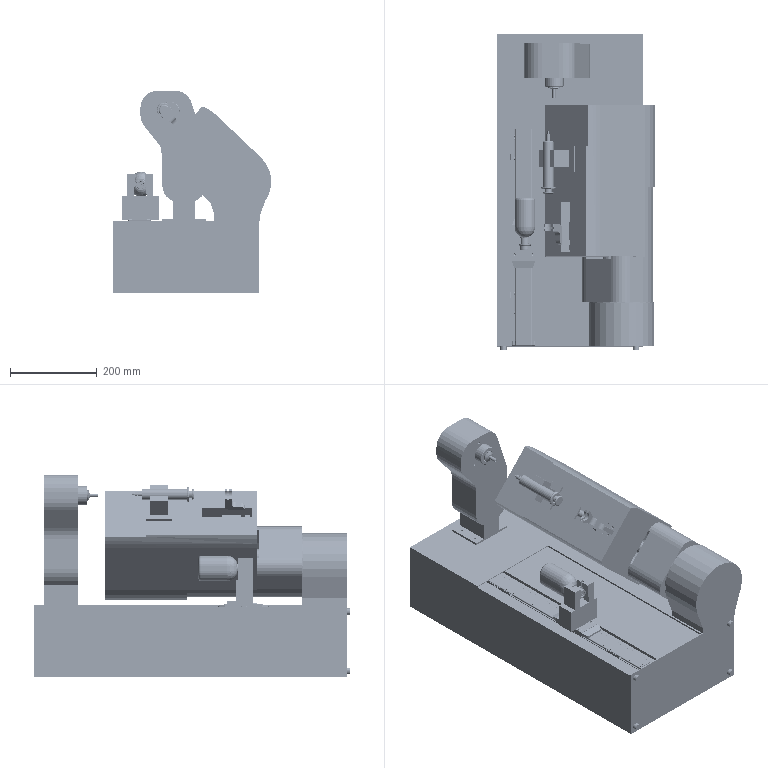Assembly | SolidWorks | mm | 70 component files | 94 solids | 5517 faces | box 364.9 x 728 x 466.99 mm | volume 10664747 mm3 | plane 2518 | cylinder 1839 | cone 608 | torus 290 | spline 142 | sphere 120 | commonest cylinder face diameters 4 x124 3.3 x122 8 x92 2 x85 4.5 x66 3 x64 5.5 x62 6 x61
Bill of materials:
1 | 1 |  | Long straight prismatic extrusion with a rectangular, double-cell slotted cross-section; looks like a T-slot framing profile.
circlips for shaft--type a small gb_GB_CONNECTING_PIECE_RING_RRA 8 | 1 |  | Thin flat open ring with a lobe on one side. A radial split passes through the lobe and has a small circular cutout across it.
Copy(10) | 1 |  | Cylindrical part made of two end hubs and a middle section with interlocking jaw or tooth blocks. It has an axial bore, and one end has a radial clamp slit. Resembles a jaw-type shaft coupling.
Copy(11) | 1 |  | Housing with a square body and a square front flange, a circular pilot boss, and a protruding cylindrical shaft with a keyway or flat. Resembles a rotary motor envelope.
Copy(2) | 1 |  | Flanged cylindrical sleeve with a through bore. The circular flange has two straight flats and six bolt holes. Resembles a flanged nut or bushing.
Copy(3) | 1 |  | Stepped cylindrical shaft: a long main diameter with reduced-diameter journals at both ends. One end has a longer journal; the other has a short double step.
Copy(4) | 1 |  | Long straight rail with a profiled cross-section, side grooves and a row of evenly spaced vertical counterbored holes along its length. Resembles a linear guide rail.
Copy(5) | 1 |  | Rectangular block with an inverted-channel underside shaped to straddle a rail, four mounting holes on top, and end caps or plates. Resembles a linear guide carriage.
Copy(6) | 1 |  | Rectangular block with a large through bore, several groups of small holes on different faces, and a shallow step or rebate along one lower edge.
Copy(7) | 1 |  | L-shaped bracket. The upright plate carries a large through hole; the base leg has two counterbored mounting holes. Resembles a shaft or bearing support bracket.
Copy(8) | 1 |  | Flat rectangular plate with one rounded corner, one large through hole near one end and two small through holes near the opposite end.
Copy(9) | 1 |  | Flat rectangular plate with one rounded corner, a large central through hole and six smaller holes of two sizes. Possibly a mounting or adapter plate.
deep groove ball bearings gb_Rolling bearings 608 GB 276-94 | 2 |  | Ring-shaped assembly that looks like a radial ball bearing: a concentric outer ring and inner ring with a row of spherical balls between them.
hex nuts, style 1-grades ab gb_GB_FASTENER_NUT_SNAB1 M4-N | 2 |  | Hexagonal nut-like prism with a central cylindrical through-bore and chamfered corners on both faces.
hexagon socket head cap screws gb_GB_FASTENER_SCREWS_HSHCS M3X8-N | 7 |  | Cap-screw-like fastener: a cylindrical head with a hexagonal socket recess and a plain cylindrical shank with a chamfered tip.
hexagon socket head cap screws gb_GB_FASTENER_SCREWS_HSHCS M4X16-N | 4 |  | Headed pin or screw-like part: a cylindrical head with a rounded top edge and a long, slender plain cylindrical shank with a chamfered end.
hexagon socket head cap screws gb_GB_FASTENER_SCREWS_HSHCS M4X8-N | 2 |  | Short cap-screw-like fastener: a cylindrical head with a hexagonal socket and a short plain cylindrical shank.
20mL - Glass Barrel | 1 | Glass | Long hollow cylindrical barrel. One end has a flange with flats; the other end has a stepped, narrow nozzle-like tip with a small axial hole. The shape resembles a syringe or cartridge barrel.
20mL - Glass Syringe Plunger | 1 | Glass | Solid stepped cylindrical rod: a thin disc-shaped end flange, a short reduced-diameter neck, and a long main cylinder with a chamfered far end. The shape resembles a plunger.
InjectionFixture | 1 |  | Prismatic block with a stepped outline, a semicircular cutout on one side and a thin plate-like flange along one edge.
_GTH5.-BC_body6^3359524133GTH5-400-BC(2) | 1 |  | Block-shaped bracket or housing: a rectangular body with a curved saddle-like channel across its top, and a thin back plate with two small holes and a larger circular opening.
GTH4-sensor_plant | 3 |  | L-shaped bent sheet-metal-style bracket. The horizontal flange has two open slots and four round holes; the vertical flange carries two stepped cylindrical pins.
GTH4-sensor | 3 |  | Rectangular body with two upright prongs that form an open U-shaped slot, an elongated base, a cylindrical rod or cable stub out one end, and a mounting tab with a small cylindrical boss. The shape resembles a slot-type sensor package.
GTH5_body3 | 1 |  | Flat plate with a T-shaped outline and rounded edges. It has a wider lower section with four counterbored holes and a narrower upper section with a step or groove near its top edge.
GTH5_body4 | 1 |  | Thick, nearly square plate with one large central circular through-hole that has a stepped/counterbored edge, and four small through-holes in two pairs near the lower corners.
GTH5-400-BC_body | 1 |  | Long straight extruded-profile body with a stepped cross-section: a wide lower base and a narrower upper section with slots along both sides near the top, end plates/caps with small fasteners, and a row of evenly spaced small holes along the length.
GTH5-400-BC_body2 | 1 |  | Very thin, long, narrow flat strip with two small holes at each end.
GTH5-400-BC_slider | 1 |  | Flat, rectangular carriage-like plate with tapered (chamfered-outline) end sections, a pattern of counterbored holes and socket-head-like fastener features on top, raised pads, and a small cylindrical stub sticking out of one side.
GTH5-50-BC_slider2 | 1 |  | Bent flat-bar bracket with a Z or joggled profile: two parallel offset legs joined by a short perpendicular web. One leg has two round through-holes.
GTH5-BC_body5 | 1 |  | U-shaped (inverted channel) cover made from a thin wall, with raised embossed lettering on the top face and a small circular boss or hole on one side wall.
M10-p1 | 1 |  | Compact rectangular block body made of several stacked segments, including one tapered section. A stepped cylindrical shaft sticks out of one face from a rectangular boss, there is a second short cylindrical stub, and a rounded rib runs along one edge.
ArmHousing | 1 |  | Solid prismatic extrusion with a keyhole/bulb-shaped profile: a circular arc top that narrows into tapered flanks and ends in a short rectangular base.
ArmHousing2 | 1 |  | Very thin flat plate with the same bulb/keyhole outline as a rounded tab: a circular top with a large concentric round hole, tapered sides, and a straight rectangular foot.
ArmHousing3 | 1 |  | Long solid prism with a rounded, teardrop/rounded-triangular cross-section. One end face has a central round hole surrounded by a ring of small holes.
DAS-15SS^ClampBlock | 1 |  | Stepped cylindrical body: a larger-diameter flange section with three axial through-holes and a smaller-diameter tubular spigot with a central bore. Two hex-bodied fittings stick out radially from the flange periphery, and there are small radial holes in the spigot.
YB-15^ClampBlock | 1 |  | Collet-like cylindrical part: a tapered head with an outward cone, three longitudinal slots splitting the head end, a central bore, plain cylindrical bands, and an externally threaded end.
FlatJawHousing | 1 |  | Thin flat plate with a bent, elongated outline: a wide rounded upper lobe angled to one side, a straighter lower section, and a narrow neck that ends in a thin T-shaped foot strip.
Housing | 1 |  | Rectangular box-shaped solid. The top face has a long recessed channel along one edge, a stepped panel line, small holes, and a stepped notch cutout at one corner. Short cylindrical studs stick out from one end face.
InjectionRodClamp | 1 |  | Bent bracket arm with an S-shaped joggle. One end is a forked or slotted tip with a semicircular notch. The other end is a rectangular mounting block with four through holes.
LiquidReagentBottle | 1 |  | Bottle-like solid of revolution: a cylindrical body with a rounded closed end, a curved shoulder, and a stepped neck with a raised collar. The end face carries concentric rings and two small circular features.
MotorHousing | 1 |  | Thin-walled shell with a D-shaped or U-shaped cross section: flat sides joined by a semicircular end. It has an offset stepped section and a rectangular window or slot in one side wall.
NeedleClampBlock | 1 |  | Thick block with the same bent, elongated outline as a lobed plate. The upper lobe has a large circular through bore with three small holes around it. A narrower neck stands on a thin base plate that has small holes.
NeedleSleeve | 1 |  | Stepped cylindrical tube: a longer section with a larger outside diameter and a shorter section with a smaller one. One end is open with a visible bore.
100Travel3872-3DDrawing | 1 |  | Housing with two parallel cylinders: a shorter cylinder and a longer main tube, joined at one end by a rounded housing block. A short tab with a cross hole sticks out from that end.
Axis | 1 |  | Slender, straight solid cylindrical rod, rendered dark. There may be small cross holes near the ends.
PushRodMotorPlatform | 1 |  | Flat circular disc with a smaller raised concentric step on one face, a central through hole, and a ring of twelve small holes around the centre. Two of the ring holes look slightly larger.
ReagentBottleClampBlock | 1 |  | Rectangular base block with two upright posts separated by a gap with curved, tapering walls. The post tops have notches. One face has two round holes, and there is a small stepped ledge at one side.
Base | 1 | 45 | Square block with chamfered corners, a central through bore, and four corner holes on the main face. A circular boss or pilot sticks out from the back. The stepped side faces carry several holes, some of which appear countersunk.
EE_SX672 | 1 |  | Rectangular block housing with an open U-shaped slot that splits it into two parallel arms. It has a pair of side mounting flanges with obround holes and four flat tab terminals, each with a round hole, along one end.
hexagon socket button head screws gb | 2 |  | Solid round shank with a dome-shaped (round) head at one end and a flat, plain end at the other.
InductionPlate | 1 | 45 | Bent flat strip shaped as a 90-degree L-bracket. It has a short top leg and a longer leg with rounded lower corners and two round through-holes.
PlanetaryReducer | 1 | 45 | Body with a square flange and a protruding cylindrical shaft. It has a square mounting flange with four corner holes, a round raised boss (pilot) around the shaft, a body with lengthwise recessed channels, and a wider square base with chamfered corners.
Turntable | 1 | 45 | Stepped cylindrical bushing with a central through-hole, a larger-diameter flange at one end, and a rectangular notch cut into the flange rim.
Mates:
1. coincident | 3359524133GTH5-400-BC(2)-1/GTH5-400-BC_slider-1 face at (334.847, 1139.269, -2179.834) dir (0, 0, 1) | ReagentBottleClampBlock-1 face at (362.347, 1094.769, -2179.834) dir (0, 0, -1)
2. distance | 3359524133GTH5-400-BC(2)-1/GTH5-400-BC_slider-1 face at (334.847, 1139.769, -2181.334) dir (0, 1, 0) | ReagentBottleClampBlock-1 face at (392.347, 1114.769, -2124.834) dir (0, 1, 0)
3. distance | ReagentBottleClampBlock-1 face at (319.847, 1074.769, -2179.834) dir (-1, 0, 0) | 3359524133GTH5-400-BC(2)-1/GTH5-400-BC_slider-1 face at (334.847, 1139.769, -2179.334) dir (-1, 0, 0)
4. lock | ReagentBottleClampBlock-1 reference at (0, 0, 0) dir (1, 0, 0) | LiquidReagentBottle-1 reference at (0, 0, 0) dir (1, 0, 0)
5. concentric | ArmHousing-1 face at (586.439, 647.868, -2092.934) dir (0, 1, 0) r 73 | RR40-1/Base-1 face at (586.439, 948, -2092.934) dir (0, -1, 0) r 47.5
6. distance | ArmHousing-1 face at (365.049, 960, -2167.934) dir (0, 1, 0) | RR40-1/InductionPlate-1 face at (594.447, 958, -2063.065) dir (0, 1, 0)
7. coincident | ArmHousing-1 edge at (586.439, 960, -2092.934) dir (0, 1, 0) r 75 | ArmHousing2-1 edge at (586.439, 960, -2092.934) dir (0, 1, 0) r 75
8. coincident | Housing-1 face at (129.525, 1580, -2182.934) dir (0, 0, 1) | ArmHousing-1 face at (365.049, 1412, -2182.934) dir (0, 0, -1)
9. coincident | Housing-1 face at (299.537, 860, -2241.334) dir (0, -1, 0) | ArmHousing-1 face at (365.049, 860, -2167.934) dir (0, -1, 0)
10. coincident | ArmHousing-1 edge at (533.489, 960, -2182.934) dir (1, 0, 0) | ArmHousing2-1 edge at (639.388, 960, -2182.934) dir (-1, 0, 0)
11. concentric | ArmHousing-1 face at (586.439, 647.868, -2092.934) dir (0, 1, 0) r 75 | ArmHousing3-1 face at (586.439, 1312, -2092.934) dir (0, -1, 0) r 73
12. parallel | Housing-1 face at (299.537, 860, -2241.334) dir (-1, 0, 0) | RR40-1/PlanetaryReducer-1 face at (564.439, 929.394, -2176.934) dir (-1, 0, 0)
13. coincident | ArmHousing2-1 face at (586.439, 962, -2092.934) dir (0, 1, 0) | ArmHousing3-1 face at (586.439, 962, -2092.934) dir (0, -1, 0)
14. parallel | ArmHousing2-1 face at (586.439, 962, -2092.934) dir (0, 1, 0) | MotorHousing-1 face at (584.807, 1067, -2032.144) dir (0, -1, 0)
15. parallel | ArmHousing3-1 face at (483.238, 1312, -2095.704) dir (-0.7258, 0, 0.6879) | 100-1/Copy(8)-1 face at (519.079, 1072, -2057.886) dir (0.7258, 0, -0.6879)
16. coincident | ArmHousing3-1 face at (483.238, 1312, -2095.704) dir (-0.7258, 0, 0.6879) | 100-1/Copy(8)-1 face at (519.079, 1072, -2057.886) dir (0.7258, 0, -0.6879)
17. concentric | ArmHousing3-1 face at (615.297, 964, -2105.562) dir (0, -1, 0) r 1.65 | PushRodMotorPlatform-1 face at (615.297, 976, -2105.562) dir (0, -1, 0) r 1.65
18. concentric | ArmHousing3-1 face at (557.104, 964, -2104.41) dir (0, -1, 0) r 1.65 | PushRodMotorPlatform-1 face at (557.104, 976, -2104.41) dir (0, -1, 0) r 1.65
19. concentric | ArmHousing3-1 face at (586.439, 1312, -2092.934) dir (0, -1, 0) r 73 | MotorHousing-1 face at (586.439, 1427, -2092.934) dir (0, -1, 0) r 78
20. coincident | PushRodMotorPlatform-1 face at (586.439, 976, -2092.934) dir (0, 1, 0) | PushRodMotor-1/100Travel3872-3DDrawing-1 face at (588.412, 976, -2097.251) dir (0, -1, 0)
21. lock | PushRodMotorPlatform-1 reference at (0, 0, 0) dir (1, 0, 0) | PushRodMotor-1/100Travel3872-3DDrawing-1 reference at (0, 0, 0) dir (1, 0, 0)
22. coincident | PushRodMotor-1/Axis-1 face at (588.412, 1411.001, -2097.251) dir (0, 1, 0) | MotorHousing-1 face at (482.645, 1411.001, -1994.567) dir (0, -1, 0)
23. coincident | MotorHousing-1 face at (512.224, 1072, -1963.357) dir (0, 1, 0) | 100-1/Copy(8)-1 face at (509.935, 1072, -2020.287) dir (0, -1, 0)
24. lock | MotorHousing-1 reference at (0, 0, 0) dir (1, 0, 0) | 100-1/Copy(8)-1 reference at (0, 0, 0) dir (1, 0, 0)
25. coincident | MotorHousing-1 face at (409.292, 860.697, -2021.086) dir (-0.7258, 0, 0.6879) | 20mL - Glass Syringe-1/InjectionFixture-1 face at (459.791, 1332, -1967.801) dir (0.7258, 0, -0.6879)
26. parallel | MotorHousing-1 face at (584.807, 1067, -2032.144) dir (0, -1, 0) | 20mL - Glass Syringe-1/InjectionFixture-1 face at (480.427, 1322, -1946.026) dir (0, 1, 0)
27. distance | 20mL - Glass Syringe-1/InjectionFixture-1 face at (480.427, 1262, -1946.026) dir (0.6879, 0, 0.7258) | MotorHousing-1 edge at (505.191, 1067, -1919.897) dir (0, 1, 0)
28. coincident | MotorHousing-1 face at (482.645, 1322, -1994.567) dir (0, 1, 0) | 20mL - Glass Syringe-1/InjectionFixture-1 face at (480.427, 1322, -1946.026) dir (0, 1, 0)
29. concentric | 100-1/Copy(6)-1 face at (489.45, 1091.461, -1987.096) dir (-0.7258, 0, 0.6879) r 3 | InjectionRodClamp-1 face at (485.821, 1091.461, -1983.657) dir (0.7258, 0, -0.6879) r 3
30. coincident | 100-1/Copy(6)-1 face at (499.081, 1146.461, -1976.934) dir (-0.7258, 0, 0.6879) | InjectionRodClamp-1 edge at (470.534, 1086.461, -2007.056) dir (0.6879, 0, 0.7258)
31. concentric | 100-1/Copy(6)-1 face at (475.693, 1106.461, -2001.613) dir (-0.7258, 0, 0.6879) r 3 | InjectionRodClamp-1 face at (472.064, 1106.461, -1998.173) dir (0.7258, 0, -0.6879) r 3
32. coincident | NeedleClampBlock-1 face at (431.234, 1505.5, -1930.507) dir (0, 1, 0) | ClampBlock-1/DAS-15SS^ClampBlock-1 face at (421.906, 1505.5, -1894.186) dir (0, -1, 0)
33. concentric | NeedleClampBlock-1 face at (431.234, 1577.5, -1930.507) dir (0, -1, 0) r 37.5 | ClampBlock-1/DAS-15SS^ClampBlock-1 face at (431.234, 1547.5, -1930.507) dir (0, 1, 0) r 37.5
34. concentric | ClampBlock-1/DAS-15SS^ClampBlock-1 face at (431.234, 1547.5, -1930.507) dir (0, 1, 0) r 22 | NeedleSleeve-1 face at (431.234, 1462, -1930.507) dir (0, -1, 0) r 4
35. distance | NeedleSleeve-1 face at (431.234, 1432, -1930.507) dir (0, -1, 0) | ClampBlock-1/YB-15^ClampBlock-1 face at (429.741, 1452, -1924.696) dir (0, -1, 0)
36. lock | Copy(2)-1 reference at (0, 0, 0) dir (1, 0, 0) | Copy(6)-1 reference at (0, 0, 0) dir (1, 0, 0)
37. concentric | Copy(2)-1 edge at (67.217, 31.308, -101.146) dir (-1, 0, 0) r 8 | Copy(3)-1 face at (-63.322, 31.308, -101.146) dir (1, 0, 0) r 8
38. lock | Copy(5)-1 reference at (0, 0, 0) dir (1, 0, 0) | Copy(6)-1 reference at (0, 0, 0) dir (1, 0, 0)
39. concentric | Copy(4)-1 face at (140.678, 6.808, -95.146) dir (-1, 0, 0) r 1.25 | Copy(5)-1 edge at (107.367, 6.808, -95.146) dir (1, 0, 0) r 1.25
40. coincident | 20mL - Glass Barrel-1 plane at (0, 0, 0) dir (0, 0, 1) | 20mL - Glass Syringe plane at (0, 0, 0) dir (0, 0, 1)
41. coincident | 20mL - Glass Barrel-1 plane at (0, 0, 0) dir (0, 1, 0) | 20mL - Glass Syringe plane at (0, 0, 0) dir (0, 1, 0)
42. coincident | 20mL - Glass Barrel-1 plane at (0, 0, 0) dir (1, 0, 0) | 20mL - Glass Syringe plane at (0, 0, 0) dir (1, 0, 0)
43. concentric | 20mL - Glass Barrel-1 face at (0, 0, 0) dir (-1, 0, 0) r 12.5 | 20mL - Glass Syringe Plunger-1 face at (-11.5, 0, 0) dir (-1, 0, 0) r 9.5
44. distance | 20mL - Glass Syringe Plunger-1 face at (108, -5.209, -5.396) dir (1, 0, 0) | 20mL - Glass Barrel-1 face at (108, 8, 0) dir (-1, 0, 0)
45. distance | GTH5-400-BC_slider-1 face at (261.231, 49, -17.539) dir (0, -1, 0) | GTH5-400-BC_body2-1 face at (540, 48.05, -15) dir (0, 1, 0)
46. coincident | GTH5-400-BC_slider-1 face at (306.731, 52.2, 25.25) dir (0, 0, 1) | GTH5-50-BC_slider2-1 face at (318.731, 48.4, 25.25) dir (0, 0, -1)
47. distance | GTH5-50-BC_slider2-1 face at (309.731, 46.4, 29.25) dir (-1, 0, 0) | GTH5-400-BC_slider-1 face at (303.231, 52.2, 25.25) dir (1, 0, 0)
48. distance | GTH5-400-BC_slider-1 face at (356.231, 60, -26.25) dir (0, 0, -1) | GTH5-400-BC_body-1 face at (540, 21.5, -18) dir (0, 0, -1)
49. concentric | 100Travel3872-3DDrawing-1 face at (0, -149.8, 347) dir (0, 0, -1) r 9.75 | Axis-1 face at (0, -149.8, 582.996) dir (0, 0, -1) r 9.75
50. coincident | Base-1 plane at (0, 0, 0) dir (0, 0, 1) | RR40 plane at (0, 0, 0) dir (0, 0, 1)
51. coincident | Base-1 plane at (0, 0, 0) dir (0, 1, 0) | RR40 plane at (0, 0, 0) dir (0, 1, 0)
52. coincident | Base-1 plane at (0, 0, 0) dir (1, 0, 0) | RR40 plane at (0, 0, 0) dir (1, 0, 0)
53. concentric | Base-1 face at (0, 0, 0) dir (0, -1, 0) r 32.5 | Turntable-1 face at (0, 45, 0) dir (0, -1, 0) r 32.5
54. coincident | Base-1 face at (32.5, 45, 0) dir (0, 1, 0) | Turntable-1 face at (32.495, 45, -0.5517) dir (0, -1, 0)
55. coincident | Turntable-1 face at (-31.902, 73, 6.042) dir (0, 1, 0) | InductionPlate-1 face at (-29.868, 73, 8.008) dir (0, -1, 0)
56. concentric | Turntable-1 face at (-33.927, 73, 4.577) dir (0, 1, 0) r 1.5 | InductionPlate-1 face at (-33.927, 75, 4.577) dir (0, 1, 0) r 1.75
57. concentric | Turntable-1 face at (-34.063, 73, -3.422) dir (0, 1, 0) r 1.5 | InductionPlate-1 face at (-34.063, 75, -3.422) dir (0, 1, 0) r 1.75
58. concentric | Turntable-1 face at (-34.063, 73, -3.422) dir (0, 1, 0) r 1.5 | hexagon socket button head screws gb-3 face at (-34.063, 55, -3.422) dir (0, 1, 0) r 3
59. coincident | InductionPlate-1 face at (-29.868, 75, 8.008) dir (0, 1, 0) | hexagon socket button head screws gb-3 face at (-34.063, 75, -3.422) dir (0, -1, 0)
60. parallel | InductionPlate-1 face at (-57.619, 72, -6.523) dir (-0.01698, 0, -0.9999) | hexagon socket button head screws gb-3 face at (-32.875, 76.22, -1.442) dir (-0.01698, 0, -0.9999)
61. concentric | Turntable-1 face at (-33.927, 73, 4.577) dir (0, 1, 0) r 1.5 | hexagon socket button head screws gb-2 face at (-33.927, 55, 4.577) dir (0, 1, 0) r 3
62. coincident | InductionPlate-1 face at (-29.868, 75, 8.008) dir (0, 1, 0) | hexagon socket button head screws gb-2 face at (-33.927, 75, 4.577) dir (0, -1, 0)
63. parallel | InductionPlate-1 face at (-57.619, 72, -6.523) dir (-0.01698, 0, -0.9999) | hexagon socket button head screws gb-2 face at (-32.739, 76.22, 6.557) dir (-0.01698, 0, -0.9999)
64. coincident | Base-1 face at (-52.5, 55, -42.5) dir (-1, 0, 0) | EE_SX672-1 face at (-52.5, 50.9, -9.5) dir (1, 0, 0)
65. distance | Base-1 face at (0, 55, 0) dir (0, 1, 0) | EE_SX672-1 face at (-52.8, 54, -13) dir (0, 1, 0)
66. coincident | EE_SX672-1 plane at (-52.5, 50.9, 0) dir (0, 0, 1) | RR40 plane at (0, 0, 0) dir (0, 0, 1)
67. concentric | Base-1 face at (45.5, 27.5, 0) dir (1, 0, 0) r 17.5 | PlanetaryReducer-1 face at (52.5, 27.5, 0) dir (1, 0, 0) r 17.5
68. coincident | Base-1 face at (52.5, 55, -42.5) dir (1, 0, 0) | PlanetaryReducer-1 face at (52.5, 27.5, 0) dir (-1, 0, 0)
69. concentric | Base-1 face at (52.5, 45.178, 17.678) dir (1, 0, 0) r 1.65 | PlanetaryReducer-1 face at (84, 45.178, 17.678) dir (-1, 0, 0) r 2.25